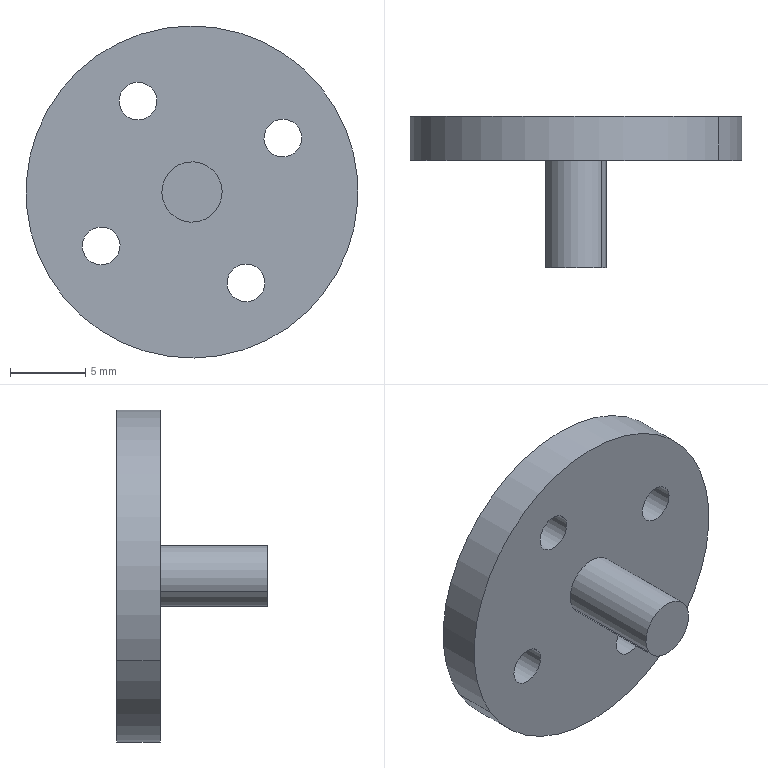Component | SolidWorks | Sheet-1 | 1 solid | 15 faces | box 22 x 10 x 22 mm | volume 1135 mm3 | cylinder 12 | plane 3 | commonest cylinder face diameters 2.5 x8 4 x2 22 x2
STEP:
#1=COLOUR_RGB('',0.7922,0.8196,0.9333);
#2=FILL_AREA_STYLE_COLOUR('',#1);
#3=FILL_AREA_STYLE('',(#2));
#4=SURFACE_STYLE_FILL_AREA(#3);
#5=SURFACE_SIDE_STYLE('',(#4));
#6=SURFACE_STYLE_USAGE(.BOTH.,#5);
#7=PRESENTATION_STYLE_ASSIGNMENT((#6));
#8=CARTESIAN_POINT('',(0.179,0.7504,2.338));
#9=VERTEX_POINT('',#8);
#10=CARTESIAN_POINT('',(0.2636,0.7504,2.388));
#11=VERTEX_POINT('',#10);
#12=CARTESIAN_POINT('',(0.2213,0.7504,2.363));
#13=DIRECTION('',(0.,1.,0.));
#14=DIRECTION('',(0.8598,0.,0.5106));
#15=AXIS2_PLACEMENT_3D('',#12,#13,#14);
#16=CIRCLE('',#15,0.04921);
#17=EDGE_CURVE('',#9,#11,#16,.T.);
#18=ORIENTED_EDGE('',*,*,#17,.F.);
#19=CARTESIAN_POINT('',(0.179,0.8646,2.338));
#20=VERTEX_POINT('',#19);
#21=CARTESIAN_POINT('',(0.179,0.4276,2.338));
#22=DIRECTION('',(0.,1.,0.));
#23=VECTOR('',#22,39.37);
#24=LINE('',#21,#23);
#25=EDGE_CURVE('',#9,#20,#24,.T.);
#26=ORIENTED_EDGE('',*,*,#25,.T.);
#27=CARTESIAN_POINT('',(0.2636,0.8646,2.388));
#28=VERTEX_POINT('',#27);
#29=CARTESIAN_POINT('',(0.2213,0.8646,2.363));
#30=DIRECTION('',(0.,1.,0.));
#31=DIRECTION('',(0.8598,0.,0.5106));
#32=AXIS2_PLACEMENT_3D('',#29,#30,#31);
#33=CIRCLE('',#32,0.04921);
#34=EDGE_CURVE('',#20,#28,#33,.T.);
#35=ORIENTED_EDGE('',*,*,#34,.T.);
#36=CARTESIAN_POINT('',(0.2636,0.4276,2.388));
#37=DIRECTION('',(0.,1.,0.));
#38=VECTOR('',#37,39.37);
#39=LINE('',#36,#38);
#40=EDGE_CURVE('',#11,#28,#39,.T.);
#41=ORIENTED_EDGE('',*,*,#40,.F.);
#42=EDGE_LOOP('',(#18,#26,#35,#41));
#43=FACE_OUTER_BOUND('',#42,.T.);
#44=CARTESIAN_POINT('',(0.2213,0.4276,2.363));
#45=DIRECTION('',(0.,1.,0.));
#46=DIRECTION('',(0.8598,0.,0.5106));
#47=AXIS2_PLACEMENT_3D('',#44,#45,#46);
#48=CYLINDRICAL_SURFACE('',#47,0.04921);
#49=ADVANCED_FACE('',(#43),#48,.F.);
#50=CARTESIAN_POINT('',(0.5566,0.7504,2.242));
#51=VERTEX_POINT('',#50);
#52=CARTESIAN_POINT('',(0.6413,0.7504,2.292));
#53=VERTEX_POINT('',#52);
#54=CARTESIAN_POINT('',(0.599,0.7504,2.267));
#55=DIRECTION('',(0.,1.,0.));
#56=DIRECTION('',(0.8598,0.,0.5106));
#57=AXIS2_PLACEMENT_3D('',#54,#55,#56);
#58=CIRCLE('',#57,0.04921);
#59=EDGE_CURVE('',#51,#53,#58,.T.);
#60=ORIENTED_EDGE('',*,*,#59,.F.);
#61=CARTESIAN_POINT('',(0.5566,0.8646,2.242));
#62=VERTEX_POINT('',#61);
#63=CARTESIAN_POINT('',(0.5566,0.4276,2.242));
#64=DIRECTION('',(0.,1.,0.));
#65=VECTOR('',#64,39.37);
#66=LINE('',#63,#65);
#67=EDGE_CURVE('',#51,#62,#66,.T.);
#68=ORIENTED_EDGE('',*,*,#67,.T.);
#69=CARTESIAN_POINT('',(0.6413,0.8646,2.292));
#70=VERTEX_POINT('',#69);
#71=CARTESIAN_POINT('',(0.599,0.8646,2.267));
#72=DIRECTION('',(0.,1.,0.));
#73=DIRECTION('',(0.8598,0.,0.5106));
#74=AXIS2_PLACEMENT_3D('',#71,#72,#73);
#75=CIRCLE('',#74,0.04921);
#76=EDGE_CURVE('',#62,#70,#75,.T.);
#77=ORIENTED_EDGE('',*,*,#76,.T.);
#78=CARTESIAN_POINT('',(0.6413,0.4276,2.292));
#79=DIRECTION('',(0.,1.,0.));
#80=VECTOR('',#79,39.37);
#81=LINE('',#78,#80);
#82=EDGE_CURVE('',#53,#70,#81,.T.);
#83=ORIENTED_EDGE('',*,*,#82,.F.);
#84=EDGE_LOOP('',(#60,#68,#77,#83));
#85=FACE_OUTER_BOUND('',#84,.T.);
#86=CARTESIAN_POINT('',(0.599,0.4276,2.267));
#87=DIRECTION('',(0.,1.,0.));
#88=DIRECTION('',(0.8598,0.,0.5106));
#89=AXIS2_PLACEMENT_3D('',#86,#87,#88);
#90=CYLINDRICAL_SURFACE('',#89,0.04921);
#91=ADVANCED_FACE('',(#85),#90,.F.);
#92=CARTESIAN_POINT('',(0.4604,0.7504,1.864));
#93=VERTEX_POINT('',#92);
#94=CARTESIAN_POINT('',(0.545,0.7504,1.914));
#95=VERTEX_POINT('',#94);
#96=CARTESIAN_POINT('',(0.5027,0.7504,1.889));
#97=DIRECTION('',(0.,1.,0.));
#98=DIRECTION('',(0.8598,0.,0.5106));
#99=AXIS2_PLACEMENT_3D('',#96,#97,#98);
#100=CIRCLE('',#99,0.04921);
#101=EDGE_CURVE('',#93,#95,#100,.T.);
#102=ORIENTED_EDGE('',*,*,#101,.F.);
#103=CARTESIAN_POINT('',(0.4604,0.8646,1.864));
#104=VERTEX_POINT('',#103);
#105=CARTESIAN_POINT('',(0.4604,0.4276,1.864));
#106=DIRECTION('',(0.,1.,0.));
#107=VECTOR('',#106,39.37);
#108=LINE('',#105,#107);
#109=EDGE_CURVE('',#93,#104,#108,.T.);
#110=ORIENTED_EDGE('',*,*,#109,.T.);
#111=CARTESIAN_POINT('',(0.545,0.8646,1.914));
#112=VERTEX_POINT('',#111);
#113=CARTESIAN_POINT('',(0.5027,0.8646,1.889));
#114=DIRECTION('',(0.,1.,0.));
#115=DIRECTION('',(0.8598,0.,0.5106));
#116=AXIS2_PLACEMENT_3D('',#113,#114,#115);
#117=CIRCLE('',#116,0.04921);
#118=EDGE_CURVE('',#104,#112,#117,.T.);
#119=ORIENTED_EDGE('',*,*,#118,.T.);
#120=CARTESIAN_POINT('',(0.545,0.4276,1.914));
#121=DIRECTION('',(0.,1.,0.));
#122=VECTOR('',#121,39.37);
#123=LINE('',#120,#122);
#124=EDGE_CURVE('',#95,#112,#123,.T.);
#125=ORIENTED_EDGE('',*,*,#124,.F.);
#126=EDGE_LOOP('',(#102,#110,#119,#125));
#127=FACE_OUTER_BOUND('',#126,.T.);
#128=CARTESIAN_POINT('',(0.5027,0.4276,1.889));
#129=DIRECTION('',(0.,1.,0.));
#130=DIRECTION('',(0.8598,0.,0.5106));
#131=AXIS2_PLACEMENT_3D('',#128,#129,#130);
#132=CYLINDRICAL_SURFACE('',#131,0.04921);
#133=ADVANCED_FACE('',(#127),#132,.F.);
#134=CARTESIAN_POINT('',(0.08272,0.7504,1.96));
#135=VERTEX_POINT('',#134);
#136=CARTESIAN_POINT('',(0.1673,0.7504,2.01));
#137=VERTEX_POINT('',#136);
#138=CARTESIAN_POINT('',(0.125,0.7504,1.985));
#139=DIRECTION('',(0.,1.,0.));
#140=DIRECTION('',(0.8598,0.,0.5106));
#141=AXIS2_PLACEMENT_3D('',#138,#139,#140);
#142=CIRCLE('',#141,0.04921);
#143=EDGE_CURVE('',#135,#137,#142,.T.);
#144=ORIENTED_EDGE('',*,*,#143,.F.);
#145=CARTESIAN_POINT('',(0.08272,0.8646,1.96));
#146=VERTEX_POINT('',#145);
#147=CARTESIAN_POINT('',(0.08272,0.4276,1.96));
#148=DIRECTION('',(0.,1.,0.));
#149=VECTOR('',#148,39.37);
#150=LINE('',#147,#149);
#151=EDGE_CURVE('',#135,#146,#150,.T.);
#152=ORIENTED_EDGE('',*,*,#151,.T.);
#153=CARTESIAN_POINT('',(0.1673,0.8646,2.01));
#154=VERTEX_POINT('',#153);
#155=CARTESIAN_POINT('',(0.125,0.8646,1.985));
#156=DIRECTION('',(0.,1.,0.));
#157=DIRECTION('',(0.8598,0.,0.5106));
#158=AXIS2_PLACEMENT_3D('',#155,#156,#157);
#159=CIRCLE('',#158,0.04921);
#160=EDGE_CURVE('',#146,#154,#159,.T.);
#161=ORIENTED_EDGE('',*,*,#160,.T.);
#162=CARTESIAN_POINT('',(0.1673,0.4276,2.01));
#163=DIRECTION('',(0.,1.,0.));
#164=VECTOR('',#163,39.37);
#165=LINE('',#162,#164);
#166=EDGE_CURVE('',#137,#154,#165,.T.);
#167=ORIENTED_EDGE('',*,*,#166,.F.);
#168=EDGE_LOOP('',(#144,#152,#161,#167));
#169=FACE_OUTER_BOUND('',#168,.T.);
#170=CARTESIAN_POINT('',(0.125,0.4276,1.985));
#171=DIRECTION('',(0.,1.,0.));
#172=DIRECTION('',(0.8598,0.,0.5106));
#173=AXIS2_PLACEMENT_3D('',#170,#171,#172);
#174=CYLINDRICAL_SURFACE('',#173,0.04921);
#175=ADVANCED_FACE('',(#169),#174,.F.);
#176=CARTESIAN_POINT('',(0.2943,0.4709,2.086));
#177=VERTEX_POINT('',#176);
#178=CARTESIAN_POINT('',(0.4297,0.4709,2.166));
#179=VERTEX_POINT('',#178);
#180=CARTESIAN_POINT('',(0.362,0.4709,2.126));
#181=DIRECTION('',(0.,-1.,0.));
#182=DIRECTION('',(-0.8598,0.,-0.5106));
#183=AXIS2_PLACEMENT_3D('',#180,#181,#182);
#184=CIRCLE('',#183,0.07874);
#185=EDGE_CURVE('',#177,#179,#184,.T.);
#186=ORIENTED_EDGE('',*,*,#185,.F.);
#187=CARTESIAN_POINT('',(0.2943,0.7504,2.086));
#188=VERTEX_POINT('',#187);
#189=CARTESIAN_POINT('',(0.2943,0.4709,2.086));
#190=DIRECTION('',(0.,1.,0.));
#191=VECTOR('',#190,39.37);
#192=LINE('',#189,#191);
#193=EDGE_CURVE('',#177,#188,#192,.T.);
#194=ORIENTED_EDGE('',*,*,#193,.T.);
#195=CARTESIAN_POINT('',(0.4297,0.7504,2.166));
#196=VERTEX_POINT('',#195);
#197=CARTESIAN_POINT('',(0.362,0.7504,2.126));
#198=DIRECTION('',(0.,-1.,0.));
#199=DIRECTION('',(0.8598,0.,0.5106));
#200=AXIS2_PLACEMENT_3D('',#197,#198,#199);
#201=CIRCLE('',#200,0.07874);
#202=EDGE_CURVE('',#188,#196,#201,.T.);
#203=ORIENTED_EDGE('',*,*,#202,.T.);
#204=CARTESIAN_POINT('',(0.4297,0.4709,2.166));
#205=DIRECTION('',(0.,1.,0.));
#206=VECTOR('',#205,39.37);
#207=LINE('',#204,#206);
#208=EDGE_CURVE('',#179,#196,#207,.T.);
#209=ORIENTED_EDGE('',*,*,#208,.F.);
#210=EDGE_LOOP('',(#186,#194,#203,#209));
#211=FACE_OUTER_BOUND('',#210,.T.);
#212=CARTESIAN_POINT('',(0.362,0.4709,2.126));
#213=DIRECTION('',(0.,1.,0.));
#214=DIRECTION('',(0.8598,0.,0.5106));
#215=AXIS2_PLACEMENT_3D('',#212,#213,#214);
#216=CYLINDRICAL_SURFACE('',#215,0.07874);
#217=ADVANCED_FACE('',(#211),#216,.T.);
#218=CARTESIAN_POINT('',(0.7344,0.8646,2.347));
#219=VERTEX_POINT('',#218);
#220=CARTESIAN_POINT('',(-0.01038,0.8646,1.905));
#221=VERTEX_POINT('',#220);
#222=CARTESIAN_POINT('',(0.362,0.8646,2.126));
#223=DIRECTION('',(0.,1.,0.));
#224=DIRECTION('',(0.8598,0.,0.5106));
#225=AXIS2_PLACEMENT_3D('',#222,#223,#224);
#226=CIRCLE('',#225,0.4331);
#227=EDGE_CURVE('',#219,#221,#226,.T.);
#228=ORIENTED_EDGE('',*,*,#227,.F.);
#229=CARTESIAN_POINT('',(0.7344,0.7504,2.347));
#230=VERTEX_POINT('',#229);
#231=CARTESIAN_POINT('',(0.7344,0.8646,2.347));
#232=DIRECTION('',(0.,-1.,0.));
#233=VECTOR('',#232,39.37);
#234=LINE('',#231,#233);
#235=EDGE_CURVE('',#219,#230,#234,.T.);
#236=ORIENTED_EDGE('',*,*,#235,.T.);
#237=CARTESIAN_POINT('',(-0.01038,0.7504,1.905));
#238=VERTEX_POINT('',#237);
#239=CARTESIAN_POINT('',(0.362,0.7504,2.126));
#240=DIRECTION('',(0.,1.,0.));
#241=DIRECTION('',(0.8598,0.,0.5106));
#242=AXIS2_PLACEMENT_3D('',#239,#240,#241);
#243=CIRCLE('',#242,0.4331);
#244=EDGE_CURVE('',#230,#238,#243,.T.);
#245=ORIENTED_EDGE('',*,*,#244,.T.);
#246=CARTESIAN_POINT('',(-0.01038,0.8646,1.905));
#247=DIRECTION('',(0.,-1.,0.));
#248=VECTOR('',#247,39.37);
#249=LINE('',#246,#248);
#250=EDGE_CURVE('',#221,#238,#249,.T.);
#251=ORIENTED_EDGE('',*,*,#250,.F.);
#252=EDGE_LOOP('',(#228,#236,#245,#251));
#253=FACE_OUTER_BOUND('',#252,.T.);
#254=CARTESIAN_POINT('',(0.362,0.8646,2.126));
#255=DIRECTION('',(0.,-1.,0.));
#256=DIRECTION('',(-0.8598,0.,-0.5106));
#257=AXIS2_PLACEMENT_3D('',#254,#255,#256);
#258=CYLINDRICAL_SURFACE('',#257,0.4331);
#259=ADVANCED_FACE('',(#253),#258,.T.);
#260=CARTESIAN_POINT('',(0.2213,0.7504,2.363));
#261=DIRECTION('',(0.,1.,0.));
#262=DIRECTION('',(0.8598,0.,0.5106));
#263=AXIS2_PLACEMENT_3D('',#260,#261,#262);
#264=CIRCLE('',#263,0.04921);
#265=EDGE_CURVE('',#11,#9,#264,.T.);
#266=ORIENTED_EDGE('',*,*,#265,.T.);
#267=ORIENTED_EDGE('',*,*,#17,.T.);
#268=EDGE_LOOP('',(#266,#267));
#269=FACE_BOUND('',#268,.T.);
#270=CARTESIAN_POINT('',(0.599,0.7504,2.267));
#271=DIRECTION('',(0.,1.,0.));
#272=DIRECTION('',(0.8598,0.,0.5106));
#273=AXIS2_PLACEMENT_3D('',#270,#271,#272);
#274=CIRCLE('',#273,0.04921);
#275=EDGE_CURVE('',#53,#51,#274,.T.);
#276=ORIENTED_EDGE('',*,*,#275,.T.);
#277=ORIENTED_EDGE('',*,*,#59,.T.);
#278=EDGE_LOOP('',(#276,#277));
#279=FACE_BOUND('',#278,.T.);
#280=CARTESIAN_POINT('',(0.5027,0.7504,1.889));
#281=DIRECTION('',(0.,1.,0.));
#282=DIRECTION('',(0.8598,0.,0.5106));
#283=AXIS2_PLACEMENT_3D('',#280,#281,#282);
#284=CIRCLE('',#283,0.04921);
#285=EDGE_CURVE('',#95,#93,#284,.T.);
#286=ORIENTED_EDGE('',*,*,#285,.T.);
#287=ORIENTED_EDGE('',*,*,#101,.T.);
#288=EDGE_LOOP('',(#286,#287));
#289=FACE_BOUND('',#288,.T.);
#290=CARTESIAN_POINT('',(0.125,0.7504,1.985));
#291=DIRECTION('',(0.,1.,0.));
#292=DIRECTION('',(0.8598,0.,0.5106));
#293=AXIS2_PLACEMENT_3D('',#290,#291,#292);
#294=CIRCLE('',#293,0.04921);
#295=EDGE_CURVE('',#137,#135,#294,.T.);
#296=ORIENTED_EDGE('',*,*,#295,.T.);
#297=ORIENTED_EDGE('',*,*,#143,.T.);
#298=EDGE_LOOP('',(#296,#297));
#299=FACE_BOUND('',#298,.T.);
#300=CARTESIAN_POINT('',(0.362,0.7504,2.126));
#301=DIRECTION('',(0.,1.,0.));
#302=DIRECTION('',(0.8598,0.,0.5106));
#303=AXIS2_PLACEMENT_3D('',#300,#301,#302);
#304=CIRCLE('',#303,0.4331);
#305=EDGE_CURVE('',#238,#230,#304,.T.);
#306=ORIENTED_EDGE('',*,*,#305,.F.);
#307=ORIENTED_EDGE('',*,*,#244,.F.);
#308=EDGE_LOOP('',(#306,#307));
#309=FACE_OUTER_BOUND('',#308,.T.);
#310=CARTESIAN_POINT('',(0.362,0.7504,2.126));
#311=DIRECTION('',(0.,-1.,0.));
#312=DIRECTION('',(0.8598,0.,0.5106));
#313=AXIS2_PLACEMENT_3D('',#310,#311,#312);
#314=CIRCLE('',#313,0.07874);
#315=EDGE_CURVE('',#196,#188,#314,.T.);
#316=ORIENTED_EDGE('',*,*,#315,.F.);
#317=ORIENTED_EDGE('',*,*,#202,.F.);
#318=EDGE_LOOP('',(#316,#317));
#319=FACE_BOUND('',#318,.T.);
#320=CARTESIAN_POINT('',(0.362,0.7504,2.126));
#321=DIRECTION('',(0.,1.,0.));
#322=DIRECTION('',(0.8598,0.,0.5106));
#323=AXIS2_PLACEMENT_3D('',#320,#321,#322);
#324=PLANE('',#323);
#325=ADVANCED_FACE('',(#269,#279,#289,#299,#309,#319),#324,.F.);
#326=ORIENTED_EDGE('',*,*,#235,.F.);
#327=CARTESIAN_POINT('',(0.362,0.8646,2.126));
#328=DIRECTION('',(0.,1.,0.));
#329=DIRECTION('',(0.8598,0.,0.5106));
#330=AXIS2_PLACEMENT_3D('',#327,#328,#329);
#331=CIRCLE('',#330,0.4331);
#332=EDGE_CURVE('',#221,#219,#331,.T.);
#333=ORIENTED_EDGE('',*,*,#332,.F.);
#334=ORIENTED_EDGE('',*,*,#250,.T.);
#335=ORIENTED_EDGE('',*,*,#305,.T.);
#336=EDGE_LOOP('',(#326,#333,#334,#335));
#337=FACE_OUTER_BOUND('',#336,.T.);
#338=CARTESIAN_POINT('',(0.362,0.8646,2.126));
#339=DIRECTION('',(0.,-1.,0.));
#340=DIRECTION('',(-0.8598,0.,-0.5106));
#341=AXIS2_PLACEMENT_3D('',#338,#339,#340);
#342=CYLINDRICAL_SURFACE('',#341,0.4331);
#343=ADVANCED_FACE('',(#337),#342,.T.);
#344=CARTESIAN_POINT('',(0.2213,0.8646,2.363));
#345=DIRECTION('',(0.,1.,0.));
#346=DIRECTION('',(0.8598,0.,0.5106));
#347=AXIS2_PLACEMENT_3D('',#344,#345,#346);
#348=CIRCLE('',#347,0.04921);
#349=EDGE_CURVE('',#28,#20,#348,.T.);
#350=ORIENTED_EDGE('',*,*,#349,.F.);
#351=ORIENTED_EDGE('',*,*,#34,.F.);
#352=EDGE_LOOP('',(#350,#351));
#353=FACE_BOUND('',#352,.T.);
#354=CARTESIAN_POINT('',(0.599,0.8646,2.267));
#355=DIRECTION('',(0.,1.,0.));
#356=DIRECTION('',(0.8598,0.,0.5106));
#357=AXIS2_PLACEMENT_3D('',#354,#355,#356);
#358=CIRCLE('',#357,0.04921);
#359=EDGE_CURVE('',#70,#62,#358,.T.);
#360=ORIENTED_EDGE('',*,*,#359,.F.);
#361=ORIENTED_EDGE('',*,*,#76,.F.);
#362=EDGE_LOOP('',(#360,#361));
#363=FACE_BOUND('',#362,.T.);
#364=CARTESIAN_POINT('',(0.5027,0.8646,1.889));
#365=DIRECTION('',(0.,1.,0.));
#366=DIRECTION('',(0.8598,0.,0.5106));
#367=AXIS2_PLACEMENT_3D('',#364,#365,#366);
#368=CIRCLE('',#367,0.04921);
#369=EDGE_CURVE('',#112,#104,#368,.T.);
#370=ORIENTED_EDGE('',*,*,#369,.F.);
#371=ORIENTED_EDGE('',*,*,#118,.F.);
#372=EDGE_LOOP('',(#370,#371));
#373=FACE_BOUND('',#372,.T.);
#374=CARTESIAN_POINT('',(0.125,0.8646,1.985));
#375=DIRECTION('',(0.,1.,0.));
#376=DIRECTION('',(0.8598,0.,0.5106));
#377=AXIS2_PLACEMENT_3D('',#374,#375,#376);
#378=CIRCLE('',#377,0.04921);
#379=EDGE_CURVE('',#154,#146,#378,.T.);
#380=ORIENTED_EDGE('',*,*,#379,.F.);
#381=ORIENTED_EDGE('',*,*,#160,.F.);
#382=EDGE_LOOP('',(#380,#381));
#383=FACE_BOUND('',#382,.T.);
#384=ORIENTED_EDGE('',*,*,#332,.T.);
#385=ORIENTED_EDGE('',*,*,#227,.T.);
#386=EDGE_LOOP('',(#384,#385));
#387=FACE_OUTER_BOUND('',#386,.T.);
#388=CARTESIAN_POINT('',(0.362,0.8646,2.126));
#389=DIRECTION('',(0.,1.,0.));
#390=DIRECTION('',(0.8598,0.,0.5106));
#391=AXIS2_PLACEMENT_3D('',#388,#389,#390);
#392=PLANE('',#391);
#393=ADVANCED_FACE('',(#353,#363,#373,#383,#387),#392,.T.);
#394=ORIENTED_EDGE('',*,*,#193,.F.);
#395=CARTESIAN_POINT('',(0.362,0.4709,2.126));
#396=DIRECTION('',(0.,-1.,0.));
#397=DIRECTION('',(-0.8598,0.,-0.5106));
#398=AXIS2_PLACEMENT_3D('',#395,#396,#397);
#399=CIRCLE('',#398,0.07874);
#400=EDGE_CURVE('',#179,#177,#399,.T.);
#401=ORIENTED_EDGE('',*,*,#400,.F.);
#402=ORIENTED_EDGE('',*,*,#208,.T.);
#403=ORIENTED_EDGE('',*,*,#315,.T.);
#404=EDGE_LOOP('',(#394,#401,#402,#403));
#405=FACE_OUTER_BOUND('',#404,.T.);
#406=CARTESIAN_POINT('',(0.362,0.4709,2.126));
#407=DIRECTION('',(0.,1.,0.));
#408=DIRECTION('',(0.8598,0.,0.5106));
#409=AXIS2_PLACEMENT_3D('',#406,#407,#408);
#410=CYLINDRICAL_SURFACE('',#409,0.07874);
#411=ADVANCED_FACE('',(#405),#410,.T.);
#412=ORIENTED_EDGE('',*,*,#400,.T.);
#413=ORIENTED_EDGE('',*,*,#185,.T.);
#414=EDGE_LOOP('',(#412,#413));
#415=FACE_OUTER_BOUND('',#414,.T.);
#416=CARTESIAN_POINT('',(0.362,0.4709,2.126));
#417=DIRECTION('',(0.,-1.,0.));
#418=DIRECTION('',(-0.8598,0.,-0.5106));
#419=AXIS2_PLACEMENT_3D('',#416,#417,#418);
#420=PLANE('',#419);
#421=ADVANCED_FACE('',(#415),#420,.T.);
#422=ORIENTED_EDGE('',*,*,#151,.F.);
#423=ORIENTED_EDGE('',*,*,#295,.F.);
#424=ORIENTED_EDGE('',*,*,#166,.T.);
#425=ORIENTED_EDGE('',*,*,#379,.T.);
#426=EDGE_LOOP('',(#422,#423,#424,#425));
#427=FACE_OUTER_BOUND('',#426,.T.);
#428=CARTESIAN_POINT('',(0.125,0.4276,1.985));
#429=DIRECTION('',(0.,1.,0.));
#430=DIRECTION('',(0.8598,0.,0.5106));
#431=AXIS2_PLACEMENT_3D('',#428,#429,#430);
#432=CYLINDRICAL_SURFACE('',#431,0.04921);
#433=ADVANCED_FACE('',(#427),#432,.F.);
#434=ORIENTED_EDGE('',*,*,#109,.F.);
#435=ORIENTED_EDGE('',*,*,#285,.F.);
#436=ORIENTED_EDGE('',*,*,#124,.T.);
#437=ORIENTED_EDGE('',*,*,#369,.T.);
#438=EDGE_LOOP('',(#434,#435,#436,#437));
#439=FACE_OUTER_BOUND('',#438,.T.);
#440=CARTESIAN_POINT('',(0.5027,0.4276,1.889));
#441=DIRECTION('',(0.,1.,0.));
#442=DIRECTION('',(0.8598,0.,0.5106));
#443=AXIS2_PLACEMENT_3D('',#440,#441,#442);
#444=CYLINDRICAL_SURFACE('',#443,0.04921);
#445=ADVANCED_FACE('',(#439),#444,.F.);
#446=ORIENTED_EDGE('',*,*,#67,.F.);
#447=ORIENTED_EDGE('',*,*,#275,.F.);
#448=ORIENTED_EDGE('',*,*,#82,.T.);
#449=ORIENTED_EDGE('',*,*,#359,.T.);
#450=EDGE_LOOP('',(#446,#447,#448,#449));
#451=FACE_OUTER_BOUND('',#450,.T.);
#452=CARTESIAN_POINT('',(0.599,0.4276,2.267));
#453=DIRECTION('',(0.,1.,0.));
#454=DIRECTION('',(0.8598,0.,0.5106));
#455=AXIS2_PLACEMENT_3D('',#452,#453,#454);
#456=CYLINDRICAL_SURFACE('',#455,0.04921);
#457=ADVANCED_FACE('',(#451),#456,.F.);
#458=ORIENTED_EDGE('',*,*,#25,.F.);
#459=ORIENTED_EDGE('',*,*,#265,.F.);
#460=ORIENTED_EDGE('',*,*,#40,.T.);
#461=ORIENTED_EDGE('',*,*,#349,.T.);
#462=EDGE_LOOP('',(#458,#459,#460,#461));
#463=FACE_OUTER_BOUND('',#462,.T.);
#464=CARTESIAN_POINT('',(0.2213,0.4276,2.363));
#465=DIRECTION('',(0.,1.,0.));
#466=DIRECTION('',(0.8598,0.,0.5106));
#467=AXIS2_PLACEMENT_3D('',#464,#465,#466);
#468=CYLINDRICAL_SURFACE('',#467,0.04921);
#469=ADVANCED_FACE('',(#463),#468,.F.);
#470=CLOSED_SHELL('',(#49,#91,#133,#175,#217,#259,#325,#343,#393,#411,#421,#433,#445,#457,#469));
#471=MANIFOLD_SOLID_BREP('',#470);
#472=STYLED_ITEM('',(#7),#471);
#473=(LENGTH_UNIT()NAMED_UNIT(*)SI_UNIT($,.METRE.));
#474=LENGTH_MEASURE_WITH_UNIT(LENGTH_MEASURE(0.0254),#473);
#475=DIMENSIONAL_EXPONENTS(1.,0.,0.,0.,0.,0.,0.);
#476=(CONVERSION_BASED_UNIT('',#474)LENGTH_UNIT()NAMED_UNIT(#475));
#477=UNCERTAINTY_MEASURE_WITH_UNIT(LENGTH_MEASURE(0.00001),#476,'','');
#478=(NAMED_UNIT(*)PLANE_ANGLE_UNIT()SI_UNIT($,.RADIAN.));
#479=(NAMED_UNIT(*)SI_UNIT($,.STERADIAN.)SOLID_ANGLE_UNIT());
#480=(GEOMETRIC_REPRESENTATION_CONTEXT(3)GLOBAL_UNCERTAINTY_ASSIGNED_CONTEXT((#477))GLOBAL_UNIT_ASSIGNED_CONTEXT((#476,#478,#479))REPRESENTATION_CONTEXT('',''));
#481=MECHANICAL_DESIGN_GEOMETRIC_PRESENTATION_REPRESENTATION('',(#472),#480);
#482=CARTESIAN_POINT('',(0.,0.,0.));
#483=DIRECTION('',(0.,0.,1.));
#484=DIRECTION('',(1.,0.,0.));
#485=AXIS2_PLACEMENT_3D('',#482,#483,#484);
#486=(LENGTH_UNIT()NAMED_UNIT(*)SI_UNIT($,.METRE.));
#487=LENGTH_MEASURE_WITH_UNIT(LENGTH_MEASURE(0.0254),#486);
#488=DIMENSIONAL_EXPONENTS(1.,0.,0.,0.,0.,0.,0.);
#489=(CONVERSION_BASED_UNIT('',#487)LENGTH_UNIT()NAMED_UNIT(#488));
#490=UNCERTAINTY_MEASURE_WITH_UNIT(LENGTH_MEASURE(0.00001),#489,'','');
#491=(NAMED_UNIT(*)PLANE_ANGLE_UNIT()SI_UNIT($,.RADIAN.));
#492=(NAMED_UNIT(*)SI_UNIT($,.STERADIAN.)SOLID_ANGLE_UNIT());
#493=(GEOMETRIC_REPRESENTATION_CONTEXT(3)GLOBAL_UNCERTAINTY_ASSIGNED_CONTEXT((#490))GLOBAL_UNIT_ASSIGNED_CONTEXT((#489,#491,#492))REPRESENTATION_CONTEXT('',''));
#494=ADVANCED_BREP_SHAPE_REPRESENTATION('',(#471,#485),#493);
#495=PRESENTATION_LAYER_ASSIGNMENT('','',(#472));